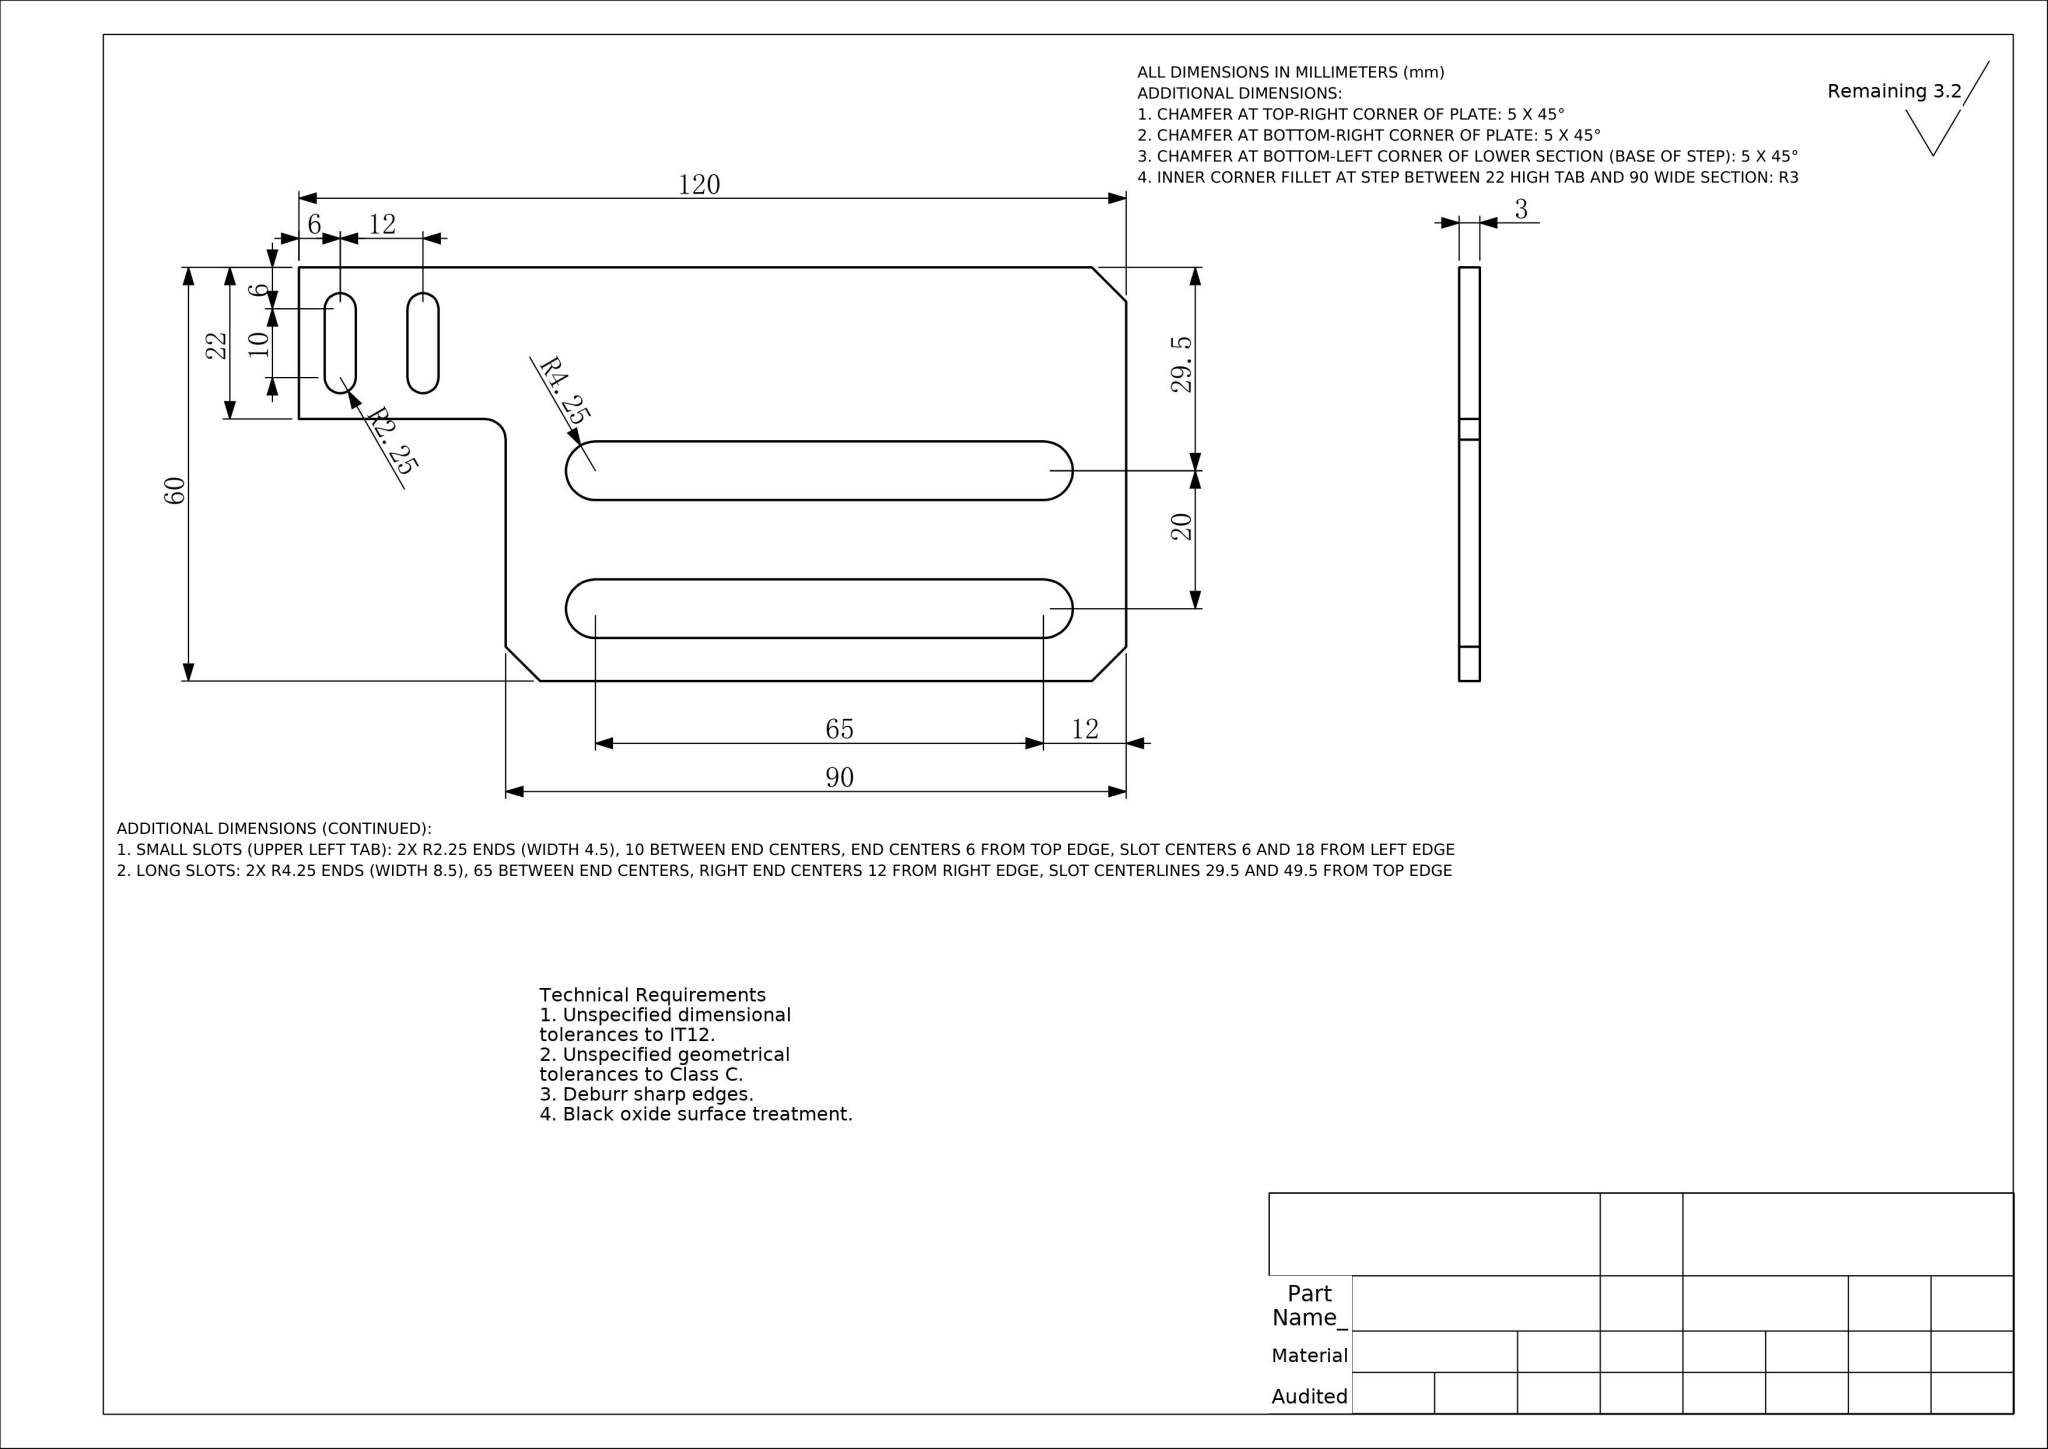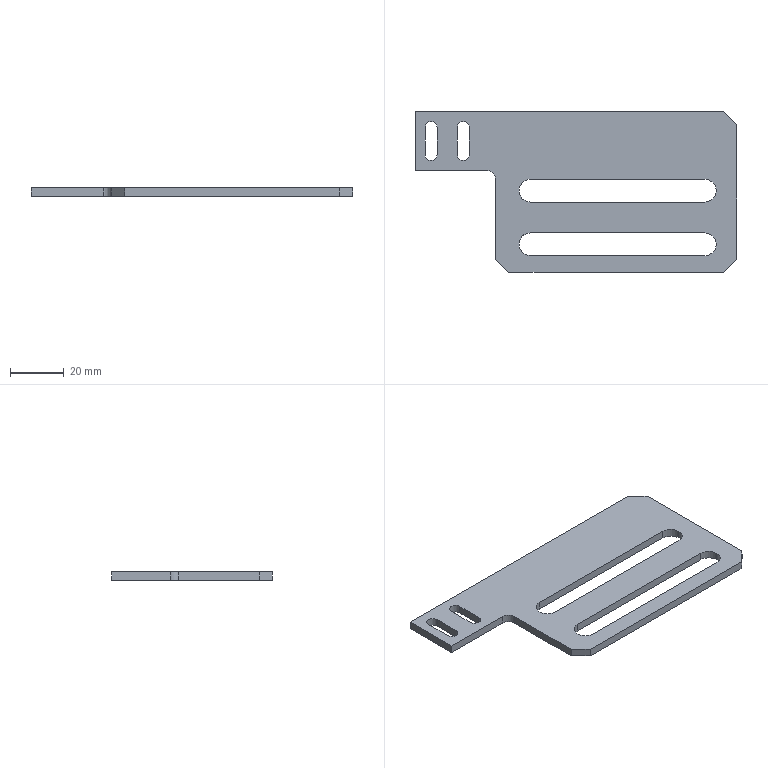Part | NX | mm | 1 solid | 30 faces | box 120 x 60 x 3 mm | volume 14052 mm3 | plane 19 | cylinder 11 | commonest cylinder face diameters 8.5 x6 4.5 x4 6 x1
STEP:
#1=COLOUR_RGB('',0.7961,0.8235,0.9373);
#2=FILL_AREA_STYLE_COLOUR('',#1);
#3=FILL_AREA_STYLE('',(#2));
#4=SURFACE_STYLE_FILL_AREA(#3);
#5=SURFACE_SIDE_STYLE('',(#4));
#6=SURFACE_STYLE_USAGE(.BOTH.,#5);
#7=PRESENTATION_STYLE_ASSIGNMENT((#6));
#8=CARTESIAN_POINT('',(108.,-45.25,-0.));
#9=VERTEX_POINT('',#8);
#10=CARTESIAN_POINT('',(112.25,-49.5,0.));
#11=VERTEX_POINT('',#10);
#12=CARTESIAN_POINT('',(108.,-49.5,0.));
#13=DIRECTION('',(0.,0.,-1.));
#14=DIRECTION('',(1.,0.,0.));
#15=AXIS2_PLACEMENT_3D('',#12,#13,#14);
#16=CIRCLE('',#15,4.25);
#17=EDGE_CURVE('',#9,#11,#16,.T.);
#18=ORIENTED_EDGE('',*,*,#17,.T.);
#19=CARTESIAN_POINT('',(112.25,-49.5,3.));
#20=VERTEX_POINT('',#19);
#21=CARTESIAN_POINT('',(112.25,-49.5,-0.001));
#22=DIRECTION('',(0.,0.,1.));
#23=VECTOR('',#22,1000.);
#24=LINE('',#21,#23);
#25=EDGE_CURVE('',#11,#20,#24,.T.);
#26=ORIENTED_EDGE('',*,*,#25,.T.);
#27=CARTESIAN_POINT('',(108.,-45.25,3.));
#28=VERTEX_POINT('',#27);
#29=CARTESIAN_POINT('',(108.,-49.5,3.));
#30=DIRECTION('',(0.,0.,1.));
#31=DIRECTION('',(-1.,0.,0.));
#32=AXIS2_PLACEMENT_3D('',#29,#30,#31);
#33=CIRCLE('',#32,4.25);
#34=EDGE_CURVE('',#20,#28,#33,.T.);
#35=ORIENTED_EDGE('',*,*,#34,.T.);
#36=CARTESIAN_POINT('',(108.,-45.25,-0.001));
#37=DIRECTION('',(0.,0.,1.));
#38=VECTOR('',#37,1000.);
#39=LINE('',#36,#38);
#40=EDGE_CURVE('',#9,#28,#39,.T.);
#41=ORIENTED_EDGE('',*,*,#40,.F.);
#42=EDGE_LOOP('',(#18,#26,#35,#41));
#43=FACE_OUTER_BOUND('',#42,.T.);
#44=CARTESIAN_POINT('',(108.,-49.5,-0.001));
#45=DIRECTION('',(0.,0.,1.));
#46=DIRECTION('',(1.,0.,0.));
#47=AXIS2_PLACEMENT_3D('',#44,#45,#46);
#48=CYLINDRICAL_SURFACE('',#47,4.25);
#49=ADVANCED_FACE('',(#43),#48,.F.);
#50=CARTESIAN_POINT('',(108.,-25.25,-0.));
#51=VERTEX_POINT('',#50);
#52=CARTESIAN_POINT('',(112.25,-29.5,0.));
#53=VERTEX_POINT('',#52);
#54=CARTESIAN_POINT('',(108.,-29.5,0.));
#55=DIRECTION('',(0.,0.,-1.));
#56=DIRECTION('',(1.,0.,0.));
#57=AXIS2_PLACEMENT_3D('',#54,#55,#56);
#58=CIRCLE('',#57,4.25);
#59=EDGE_CURVE('',#51,#53,#58,.T.);
#60=ORIENTED_EDGE('',*,*,#59,.T.);
#61=CARTESIAN_POINT('',(112.25,-29.5,3.));
#62=VERTEX_POINT('',#61);
#63=CARTESIAN_POINT('',(112.25,-29.5,-0.001));
#64=DIRECTION('',(0.,0.,1.));
#65=VECTOR('',#64,1000.);
#66=LINE('',#63,#65);
#67=EDGE_CURVE('',#53,#62,#66,.T.);
#68=ORIENTED_EDGE('',*,*,#67,.T.);
#69=CARTESIAN_POINT('',(108.,-25.25,3.));
#70=VERTEX_POINT('',#69);
#71=CARTESIAN_POINT('',(108.,-29.5,3.));
#72=DIRECTION('',(0.,0.,1.));
#73=DIRECTION('',(-1.,0.,0.));
#74=AXIS2_PLACEMENT_3D('',#71,#72,#73);
#75=CIRCLE('',#74,4.25);
#76=EDGE_CURVE('',#62,#70,#75,.T.);
#77=ORIENTED_EDGE('',*,*,#76,.T.);
#78=CARTESIAN_POINT('',(108.,-25.25,-0.001));
#79=DIRECTION('',(0.,0.,1.));
#80=VECTOR('',#79,1000.);
#81=LINE('',#78,#80);
#82=EDGE_CURVE('',#51,#70,#81,.T.);
#83=ORIENTED_EDGE('',*,*,#82,.F.);
#84=EDGE_LOOP('',(#60,#68,#77,#83));
#85=FACE_OUTER_BOUND('',#84,.T.);
#86=CARTESIAN_POINT('',(108.,-29.5,-0.001));
#87=DIRECTION('',(0.,0.,1.));
#88=DIRECTION('',(1.,0.,0.));
#89=AXIS2_PLACEMENT_3D('',#86,#87,#88);
#90=CYLINDRICAL_SURFACE('',#89,4.25);
#91=ADVANCED_FACE('',(#85),#90,.F.);
#92=CARTESIAN_POINT('',(0.,0.,0.));
#93=VERTEX_POINT('',#92);
#94=CARTESIAN_POINT('',(0.,-22.,0.));
#95=VERTEX_POINT('',#94);
#96=CARTESIAN_POINT('',(0.,0.,0.));
#97=DIRECTION('',(0.,-1.,0.));
#98=VECTOR('',#97,1000.);
#99=LINE('',#96,#98);
#100=EDGE_CURVE('',#93,#95,#99,.T.);
#101=ORIENTED_EDGE('',*,*,#100,.T.);
#102=CARTESIAN_POINT('',(0.,-22.,3.));
#103=VERTEX_POINT('',#102);
#104=CARTESIAN_POINT('',(0.,-22.,3.));
#105=DIRECTION('',(0.,0.,-1.));
#106=VECTOR('',#105,1000.);
#107=LINE('',#104,#106);
#108=EDGE_CURVE('',#103,#95,#107,.T.);
#109=ORIENTED_EDGE('',*,*,#108,.F.);
#110=CARTESIAN_POINT('',(0.,0.,3.));
#111=VERTEX_POINT('',#110);
#112=CARTESIAN_POINT('',(0.,0.,3.));
#113=DIRECTION('',(0.,-1.,0.));
#114=VECTOR('',#113,1000.);
#115=LINE('',#112,#114);
#116=EDGE_CURVE('',#111,#103,#115,.T.);
#117=ORIENTED_EDGE('',*,*,#116,.F.);
#118=CARTESIAN_POINT('',(0.,0.,3.));
#119=DIRECTION('',(0.,0.,-1.));
#120=VECTOR('',#119,1000.);
#121=LINE('',#118,#120);
#122=EDGE_CURVE('',#111,#93,#121,.T.);
#123=ORIENTED_EDGE('',*,*,#122,.T.);
#124=EDGE_LOOP('',(#101,#109,#117,#123));
#125=FACE_OUTER_BOUND('',#124,.T.);
#126=CARTESIAN_POINT('',(0.,0.,3.));
#127=DIRECTION('',(1.,0.,0.));
#128=DIRECTION('',(-0.,1.,0.));
#129=AXIS2_PLACEMENT_3D('',#126,#127,#128);
#130=PLANE('',#129);
#131=ADVANCED_FACE('',(#125),#130,.F.);
#132=CARTESIAN_POINT('',(27.,-22.,0.));
#133=VERTEX_POINT('',#132);
#134=CARTESIAN_POINT('',(0.,-22.,0.));
#135=DIRECTION('',(1.,-0.,0.));
#136=VECTOR('',#135,1000.);
#137=LINE('',#134,#136);
#138=EDGE_CURVE('',#95,#133,#137,.T.);
#139=ORIENTED_EDGE('',*,*,#138,.T.);
#140=CARTESIAN_POINT('',(27.,-22.,3.));
#141=VERTEX_POINT('',#140);
#142=CARTESIAN_POINT('',(27.,-22.,3.));
#143=DIRECTION('',(0.,0.,-1.));
#144=VECTOR('',#143,1000.);
#145=LINE('',#142,#144);
#146=EDGE_CURVE('',#141,#133,#145,.T.);
#147=ORIENTED_EDGE('',*,*,#146,.F.);
#148=CARTESIAN_POINT('',(0.,-22.,3.));
#149=DIRECTION('',(1.,-0.,0.));
#150=VECTOR('',#149,1000.);
#151=LINE('',#148,#150);
#152=EDGE_CURVE('',#103,#141,#151,.T.);
#153=ORIENTED_EDGE('',*,*,#152,.F.);
#154=ORIENTED_EDGE('',*,*,#108,.T.);
#155=EDGE_LOOP('',(#139,#147,#153,#154));
#156=FACE_OUTER_BOUND('',#155,.T.);
#157=CARTESIAN_POINT('',(0.,-22.,3.));
#158=DIRECTION('',(0.,1.,0.));
#159=DIRECTION('',(-1.,0.,0.));
#160=AXIS2_PLACEMENT_3D('',#157,#158,#159);
#161=PLANE('',#160);
#162=ADVANCED_FACE('',(#156),#161,.F.);
#163=CARTESIAN_POINT('',(30.,-25.,0.));
#164=VERTEX_POINT('',#163);
#165=CARTESIAN_POINT('',(27.,-25.,0.));
#166=DIRECTION('',(0.,0.,-1.));
#167=DIRECTION('',(1.,0.,0.));
#168=AXIS2_PLACEMENT_3D('',#165,#166,#167);
#169=CIRCLE('',#168,3.);
#170=EDGE_CURVE('',#133,#164,#169,.T.);
#171=ORIENTED_EDGE('',*,*,#170,.T.);
#172=CARTESIAN_POINT('',(30.,-25.,3.));
#173=VERTEX_POINT('',#172);
#174=CARTESIAN_POINT('',(30.,-25.,3.));
#175=DIRECTION('',(0.,0.,-1.));
#176=VECTOR('',#175,1000.);
#177=LINE('',#174,#176);
#178=EDGE_CURVE('',#173,#164,#177,.T.);
#179=ORIENTED_EDGE('',*,*,#178,.F.);
#180=CARTESIAN_POINT('',(27.,-25.,3.));
#181=DIRECTION('',(0.,0.,-1.));
#182=DIRECTION('',(1.,0.,0.));
#183=AXIS2_PLACEMENT_3D('',#180,#181,#182);
#184=CIRCLE('',#183,3.);
#185=EDGE_CURVE('',#141,#173,#184,.T.);
#186=ORIENTED_EDGE('',*,*,#185,.F.);
#187=ORIENTED_EDGE('',*,*,#146,.T.);
#188=EDGE_LOOP('',(#171,#179,#186,#187));
#189=FACE_OUTER_BOUND('',#188,.T.);
#190=CARTESIAN_POINT('',(27.,-25.,3.));
#191=DIRECTION('',(0.,0.,-1.));
#192=DIRECTION('',(-1.,0.,0.));
#193=AXIS2_PLACEMENT_3D('',#190,#191,#192);
#194=CYLINDRICAL_SURFACE('',#193,3.);
#195=ADVANCED_FACE('',(#189),#194,.F.);
#196=CARTESIAN_POINT('',(30.,-55.,0.));
#197=VERTEX_POINT('',#196);
#198=CARTESIAN_POINT('',(30.,-60.,0.));
#199=DIRECTION('',(0.,-1.,0.));
#200=VECTOR('',#199,1000.);
#201=LINE('',#198,#200);
#202=EDGE_CURVE('',#164,#197,#201,.T.);
#203=ORIENTED_EDGE('',*,*,#202,.T.);
#204=CARTESIAN_POINT('',(30.,-55.,3.));
#205=VERTEX_POINT('',#204);
#206=CARTESIAN_POINT('',(30.,-55.,3.));
#207=DIRECTION('',(0.,0.,1.));
#208=VECTOR('',#207,1000.);
#209=LINE('',#206,#208);
#210=EDGE_CURVE('',#197,#205,#209,.T.);
#211=ORIENTED_EDGE('',*,*,#210,.T.);
#212=CARTESIAN_POINT('',(30.,-60.,3.));
#213=DIRECTION('',(0.,-1.,0.));
#214=VECTOR('',#213,1000.);
#215=LINE('',#212,#214);
#216=EDGE_CURVE('',#173,#205,#215,.T.);
#217=ORIENTED_EDGE('',*,*,#216,.F.);
#218=ORIENTED_EDGE('',*,*,#178,.T.);
#219=EDGE_LOOP('',(#203,#211,#217,#218));
#220=FACE_OUTER_BOUND('',#219,.T.);
#221=CARTESIAN_POINT('',(30.,-60.,3.));
#222=DIRECTION('',(1.,0.,0.));
#223=DIRECTION('',(0.,0.,-1.));
#224=AXIS2_PLACEMENT_3D('',#221,#222,#223);
#225=PLANE('',#224);
#226=ADVANCED_FACE('',(#220),#225,.F.);
#227=CARTESIAN_POINT('',(35.,-60.,3.));
#228=VERTEX_POINT('',#227);
#229=CARTESIAN_POINT('',(115.,-60.,3.));
#230=VERTEX_POINT('',#229);
#231=CARTESIAN_POINT('',(30.,-60.,3.));
#232=DIRECTION('',(1.,0.,0.));
#233=VECTOR('',#232,1000.);
#234=LINE('',#231,#233);
#235=EDGE_CURVE('',#228,#230,#234,.T.);
#236=ORIENTED_EDGE('',*,*,#235,.F.);
#237=CARTESIAN_POINT('',(35.,-60.,0.));
#238=VERTEX_POINT('',#237);
#239=CARTESIAN_POINT('',(35.,-60.,3.));
#240=DIRECTION('',(0.,0.,-1.));
#241=VECTOR('',#240,1000.);
#242=LINE('',#239,#241);
#243=EDGE_CURVE('',#228,#238,#242,.T.);
#244=ORIENTED_EDGE('',*,*,#243,.T.);
#245=CARTESIAN_POINT('',(115.,-60.,0.));
#246=VERTEX_POINT('',#245);
#247=CARTESIAN_POINT('',(30.,-60.,0.));
#248=DIRECTION('',(1.,0.,0.));
#249=VECTOR('',#248,1000.);
#250=LINE('',#247,#249);
#251=EDGE_CURVE('',#238,#246,#250,.T.);
#252=ORIENTED_EDGE('',*,*,#251,.T.);
#253=CARTESIAN_POINT('',(115.,-60.,3.));
#254=DIRECTION('',(0.,0.,1.));
#255=VECTOR('',#254,1000.);
#256=LINE('',#253,#255);
#257=EDGE_CURVE('',#246,#230,#256,.T.);
#258=ORIENTED_EDGE('',*,*,#257,.T.);
#259=EDGE_LOOP('',(#236,#244,#252,#258));
#260=FACE_OUTER_BOUND('',#259,.T.);
#261=CARTESIAN_POINT('',(30.,-60.,3.));
#262=DIRECTION('',(0.,1.,0.));
#263=DIRECTION('',(0.,0.,1.));
#264=AXIS2_PLACEMENT_3D('',#261,#262,#263);
#265=PLANE('',#264);
#266=ADVANCED_FACE('',(#260),#265,.F.);
#267=CARTESIAN_POINT('',(120.,-55.,3.));
#268=VERTEX_POINT('',#267);
#269=CARTESIAN_POINT('',(120.,-5.,3.));
#270=VERTEX_POINT('',#269);
#271=CARTESIAN_POINT('',(120.,0.,3.));
#272=DIRECTION('',(-0.,1.,0.));
#273=VECTOR('',#272,1000.);
#274=LINE('',#271,#273);
#275=EDGE_CURVE('',#268,#270,#274,.T.);
#276=ORIENTED_EDGE('',*,*,#275,.F.);
#277=CARTESIAN_POINT('',(120.,-55.,0.));
#278=VERTEX_POINT('',#277);
#279=CARTESIAN_POINT('',(120.,-55.,3.));
#280=DIRECTION('',(0.,0.,-1.));
#281=VECTOR('',#280,1000.);
#282=LINE('',#279,#281);
#283=EDGE_CURVE('',#268,#278,#282,.T.);
#284=ORIENTED_EDGE('',*,*,#283,.T.);
#285=CARTESIAN_POINT('',(120.,-5.,0.));
#286=VERTEX_POINT('',#285);
#287=CARTESIAN_POINT('',(120.,0.,0.));
#288=DIRECTION('',(-0.,1.,0.));
#289=VECTOR('',#288,1000.);
#290=LINE('',#287,#289);
#291=EDGE_CURVE('',#278,#286,#290,.T.);
#292=ORIENTED_EDGE('',*,*,#291,.T.);
#293=CARTESIAN_POINT('',(120.,-5.,3.));
#294=DIRECTION('',(0.,0.,1.));
#295=VECTOR('',#294,1000.);
#296=LINE('',#293,#295);
#297=EDGE_CURVE('',#286,#270,#296,.T.);
#298=ORIENTED_EDGE('',*,*,#297,.T.);
#299=EDGE_LOOP('',(#276,#284,#292,#298));
#300=FACE_OUTER_BOUND('',#299,.T.);
#301=CARTESIAN_POINT('',(120.,0.,3.));
#302=DIRECTION('',(-1.,-0.,0.));
#303=DIRECTION('',(0.,-1.,0.));
#304=AXIS2_PLACEMENT_3D('',#301,#302,#303);
#305=PLANE('',#304);
#306=ADVANCED_FACE('',(#300),#305,.F.);
#307=CARTESIAN_POINT('',(115.,0.,3.));
#308=VERTEX_POINT('',#307);
#309=CARTESIAN_POINT('',(0.,0.,3.));
#310=DIRECTION('',(-1.,0.,0.));
#311=VECTOR('',#310,1000.);
#312=LINE('',#309,#311);
#313=EDGE_CURVE('',#308,#111,#312,.T.);
#314=ORIENTED_EDGE('',*,*,#313,.F.);
#315=CARTESIAN_POINT('',(115.,0.,0.));
#316=VERTEX_POINT('',#315);
#317=CARTESIAN_POINT('',(115.,0.,3.));
#318=DIRECTION('',(0.,0.,-1.));
#319=VECTOR('',#318,1000.);
#320=LINE('',#317,#319);
#321=EDGE_CURVE('',#308,#316,#320,.T.);
#322=ORIENTED_EDGE('',*,*,#321,.T.);
#323=CARTESIAN_POINT('',(0.,0.,0.));
#324=DIRECTION('',(-1.,0.,0.));
#325=VECTOR('',#324,1000.);
#326=LINE('',#323,#325);
#327=EDGE_CURVE('',#316,#93,#326,.T.);
#328=ORIENTED_EDGE('',*,*,#327,.T.);
#329=ORIENTED_EDGE('',*,*,#122,.F.);
#330=EDGE_LOOP('',(#314,#322,#328,#329));
#331=FACE_OUTER_BOUND('',#330,.T.);
#332=CARTESIAN_POINT('',(0.,0.,3.));
#333=DIRECTION('',(0.,-1.,0.));
#334=DIRECTION('',(0.,0.,-1.));
#335=AXIS2_PLACEMENT_3D('',#332,#333,#334);
#336=PLANE('',#335);
#337=ADVANCED_FACE('',(#331),#336,.F.);
#338=CARTESIAN_POINT('',(20.25,-6.,3.));
#339=VERTEX_POINT('',#338);
#340=CARTESIAN_POINT('',(15.75,-6.,3.));
#341=VERTEX_POINT('',#340);
#342=CARTESIAN_POINT('',(18.,-6.,3.));
#343=DIRECTION('',(0.,0.,1.));
#344=DIRECTION('',(-1.,0.,0.));
#345=AXIS2_PLACEMENT_3D('',#342,#343,#344);
#346=CIRCLE('',#345,2.25);
#347=EDGE_CURVE('',#339,#341,#346,.T.);
#348=ORIENTED_EDGE('',*,*,#347,.F.);
#349=CARTESIAN_POINT('',(20.25,-16.,3.));
#350=VERTEX_POINT('',#349);
#351=CARTESIAN_POINT('',(20.25,-6.,3.));
#352=DIRECTION('',(0.,1.,0.));
#353=VECTOR('',#352,1000.);
#354=LINE('',#351,#353);
#355=EDGE_CURVE('',#350,#339,#354,.T.);
#356=ORIENTED_EDGE('',*,*,#355,.F.);
#357=CARTESIAN_POINT('',(15.75,-16.,3.));
#358=VERTEX_POINT('',#357);
#359=CARTESIAN_POINT('',(18.,-16.,3.));
#360=DIRECTION('',(0.,0.,1.));
#361=DIRECTION('',(1.,0.,0.));
#362=AXIS2_PLACEMENT_3D('',#359,#360,#361);
#363=CIRCLE('',#362,2.25);
#364=EDGE_CURVE('',#358,#350,#363,.T.);
#365=ORIENTED_EDGE('',*,*,#364,.F.);
#366=CARTESIAN_POINT('',(15.75,-6.,3.));
#367=DIRECTION('',(-0.,-1.,0.));
#368=VECTOR('',#367,1000.);
#369=LINE('',#366,#368);
#370=EDGE_CURVE('',#341,#358,#369,.T.);
#371=ORIENTED_EDGE('',*,*,#370,.F.);
#372=EDGE_LOOP('',(#348,#356,#365,#371));
#373=FACE_BOUND('',#372,.T.);
#374=CARTESIAN_POINT('',(8.25,-6.,3.));
#375=VERTEX_POINT('',#374);
#376=CARTESIAN_POINT('',(3.75,-6.,3.));
#377=VERTEX_POINT('',#376);
#378=CARTESIAN_POINT('',(6.,-6.,3.));
#379=DIRECTION('',(0.,0.,1.));
#380=DIRECTION('',(-1.,0.,0.));
#381=AXIS2_PLACEMENT_3D('',#378,#379,#380);
#382=CIRCLE('',#381,2.25);
#383=EDGE_CURVE('',#375,#377,#382,.T.);
#384=ORIENTED_EDGE('',*,*,#383,.F.);
#385=CARTESIAN_POINT('',(8.25,-16.,3.));
#386=VERTEX_POINT('',#385);
#387=CARTESIAN_POINT('',(8.25,-6.,3.));
#388=DIRECTION('',(0.,1.,0.));
#389=VECTOR('',#388,1000.);
#390=LINE('',#387,#389);
#391=EDGE_CURVE('',#386,#375,#390,.T.);
#392=ORIENTED_EDGE('',*,*,#391,.F.);
#393=CARTESIAN_POINT('',(3.75,-16.,3.));
#394=VERTEX_POINT('',#393);
#395=CARTESIAN_POINT('',(6.,-16.,3.));
#396=DIRECTION('',(0.,0.,1.));
#397=DIRECTION('',(1.,0.,0.));
#398=AXIS2_PLACEMENT_3D('',#395,#396,#397);
#399=CIRCLE('',#398,2.25);
#400=EDGE_CURVE('',#394,#386,#399,.T.);
#401=ORIENTED_EDGE('',*,*,#400,.F.);
#402=CARTESIAN_POINT('',(3.75,-6.,3.));
#403=DIRECTION('',(0.,-1.,0.));
#404=VECTOR('',#403,1000.);
#405=LINE('',#402,#404);
#406=EDGE_CURVE('',#377,#394,#405,.T.);
#407=ORIENTED_EDGE('',*,*,#406,.F.);
#408=EDGE_LOOP('',(#384,#392,#401,#407));
#409=FACE_BOUND('',#408,.T.);
#410=CARTESIAN_POINT('',(43.,-45.25,3.));
#411=VERTEX_POINT('',#410);
#412=CARTESIAN_POINT('',(43.,-53.75,3.));
#413=VERTEX_POINT('',#412);
#414=CARTESIAN_POINT('',(43.,-49.5,3.));
#415=DIRECTION('',(0.,0.,1.));
#416=DIRECTION('',(1.,0.,0.));
#417=AXIS2_PLACEMENT_3D('',#414,#415,#416);
#418=CIRCLE('',#417,4.25);
#419=EDGE_CURVE('',#411,#413,#418,.T.);
#420=ORIENTED_EDGE('',*,*,#419,.F.);
#421=CARTESIAN_POINT('',(43.,-45.25,3.));
#422=DIRECTION('',(-1.,0.,0.));
#423=VECTOR('',#422,1000.);
#424=LINE('',#421,#423);
#425=EDGE_CURVE('',#28,#411,#424,.T.);
#426=ORIENTED_EDGE('',*,*,#425,.F.);
#427=ORIENTED_EDGE('',*,*,#34,.F.);
#428=CARTESIAN_POINT('',(108.,-53.75,3.));
#429=VERTEX_POINT('',#428);
#430=CARTESIAN_POINT('',(108.,-49.5,3.));
#431=DIRECTION('',(0.,0.,1.));
#432=DIRECTION('',(-1.,0.,0.));
#433=AXIS2_PLACEMENT_3D('',#430,#431,#432);
#434=CIRCLE('',#433,4.25);
#435=EDGE_CURVE('',#429,#20,#434,.T.);
#436=ORIENTED_EDGE('',*,*,#435,.F.);
#437=CARTESIAN_POINT('',(43.,-53.75,3.));
#438=DIRECTION('',(1.,0.,0.));
#439=VECTOR('',#438,1000.);
#440=LINE('',#437,#439);
#441=EDGE_CURVE('',#413,#429,#440,.T.);
#442=ORIENTED_EDGE('',*,*,#441,.F.);
#443=EDGE_LOOP('',(#420,#426,#427,#436,#442));
#444=FACE_BOUND('',#443,.T.);
#445=CARTESIAN_POINT('',(43.,-25.25,3.));
#446=VERTEX_POINT('',#445);
#447=CARTESIAN_POINT('',(43.,-33.75,3.));
#448=VERTEX_POINT('',#447);
#449=CARTESIAN_POINT('',(43.,-29.5,3.));
#450=DIRECTION('',(0.,0.,1.));
#451=DIRECTION('',(1.,0.,0.));
#452=AXIS2_PLACEMENT_3D('',#449,#450,#451);
#453=CIRCLE('',#452,4.25);
#454=EDGE_CURVE('',#446,#448,#453,.T.);
#455=ORIENTED_EDGE('',*,*,#454,.F.);
#456=CARTESIAN_POINT('',(43.,-25.25,3.));
#457=DIRECTION('',(-1.,0.,0.));
#458=VECTOR('',#457,1000.);
#459=LINE('',#456,#458);
#460=EDGE_CURVE('',#70,#446,#459,.T.);
#461=ORIENTED_EDGE('',*,*,#460,.F.);
#462=ORIENTED_EDGE('',*,*,#76,.F.);
#463=CARTESIAN_POINT('',(108.,-33.75,3.));
#464=VERTEX_POINT('',#463);
#465=CARTESIAN_POINT('',(108.,-29.5,3.));
#466=DIRECTION('',(0.,0.,1.));
#467=DIRECTION('',(-1.,0.,0.));
#468=AXIS2_PLACEMENT_3D('',#465,#466,#467);
#469=CIRCLE('',#468,4.25);
#470=EDGE_CURVE('',#464,#62,#469,.T.);
#471=ORIENTED_EDGE('',*,*,#470,.F.);
#472=CARTESIAN_POINT('',(43.,-33.75,3.));
#473=DIRECTION('',(1.,0.,0.));
#474=VECTOR('',#473,1000.);
#475=LINE('',#472,#474);
#476=EDGE_CURVE('',#448,#464,#475,.T.);
#477=ORIENTED_EDGE('',*,*,#476,.F.);
#478=EDGE_LOOP('',(#455,#461,#462,#471,#477));
#479=FACE_BOUND('',#478,.T.);
#480=ORIENTED_EDGE('',*,*,#216,.T.);
#481=CARTESIAN_POINT('',(13.5,-38.5,3.));
#482=DIRECTION('',(0.7071,-0.7071,0.));
#483=VECTOR('',#482,1000.);
#484=LINE('',#481,#483);
#485=EDGE_CURVE('',#205,#228,#484,.T.);
#486=ORIENTED_EDGE('',*,*,#485,.T.);
#487=ORIENTED_EDGE('',*,*,#235,.T.);
#488=CARTESIAN_POINT('',(88.5,-86.5,3.));
#489=DIRECTION('',(0.7071,0.7071,0.));
#490=VECTOR('',#489,1000.);
#491=LINE('',#488,#490);
#492=EDGE_CURVE('',#230,#268,#491,.T.);
#493=ORIENTED_EDGE('',*,*,#492,.T.);
#494=ORIENTED_EDGE('',*,*,#275,.T.);
#495=CARTESIAN_POINT('',(83.5,31.5,3.));
#496=DIRECTION('',(-0.7071,0.7071,0.));
#497=VECTOR('',#496,1000.);
#498=LINE('',#495,#497);
#499=EDGE_CURVE('',#270,#308,#498,.T.);
#500=ORIENTED_EDGE('',*,*,#499,.T.);
#501=ORIENTED_EDGE('',*,*,#313,.T.);
#502=ORIENTED_EDGE('',*,*,#116,.T.);
#503=ORIENTED_EDGE('',*,*,#152,.T.);
#504=ORIENTED_EDGE('',*,*,#185,.T.);
#505=EDGE_LOOP('',(#480,#486,#487,#493,#494,#500,#501,#502,#503,#504));
#506=FACE_OUTER_BOUND('',#505,.T.);
#507=CARTESIAN_POINT('',(27.,-25.,3.));
#508=DIRECTION('',(0.,0.,1.));
#509=DIRECTION('',(1.,0.,0.));
#510=AXIS2_PLACEMENT_3D('',#507,#508,#509);
#511=PLANE('',#510);
#512=ADVANCED_FACE('',(#373,#409,#444,#479,#506),#511,.T.);
#513=CARTESIAN_POINT('',(20.25,-6.,-0.));
#514=VERTEX_POINT('',#513);
#515=CARTESIAN_POINT('',(20.25,-16.,-0.));
#516=VERTEX_POINT('',#515);
#517=CARTESIAN_POINT('',(20.25,-6.,0.));
#518=DIRECTION('',(0.,-1.,0.));
#519=VECTOR('',#518,1000.);
#520=LINE('',#517,#519);
#521=EDGE_CURVE('',#514,#516,#520,.T.);
#522=ORIENTED_EDGE('',*,*,#521,.F.);
#523=CARTESIAN_POINT('',(15.75,-6.,0.));
#524=VERTEX_POINT('',#523);
#525=CARTESIAN_POINT('',(18.,-6.,0.));
#526=DIRECTION('',(0.,0.,-1.));
#527=DIRECTION('',(1.,0.,0.));
#528=AXIS2_PLACEMENT_3D('',#525,#526,#527);
#529=CIRCLE('',#528,2.25);
#530=EDGE_CURVE('',#524,#514,#529,.T.);
#531=ORIENTED_EDGE('',*,*,#530,.F.);
#532=CARTESIAN_POINT('',(15.75,-16.,0.));
#533=VERTEX_POINT('',#532);
#534=CARTESIAN_POINT('',(15.75,-6.,0.));
#535=DIRECTION('',(0.,1.,0.));
#536=VECTOR('',#535,1000.);
#537=LINE('',#534,#536);
#538=EDGE_CURVE('',#533,#524,#537,.T.);
#539=ORIENTED_EDGE('',*,*,#538,.F.);
#540=CARTESIAN_POINT('',(18.,-16.,0.));
#541=DIRECTION('',(0.,0.,-1.));
#542=DIRECTION('',(1.,0.,0.));
#543=AXIS2_PLACEMENT_3D('',#540,#541,#542);
#544=CIRCLE('',#543,2.25);
#545=EDGE_CURVE('',#516,#533,#544,.T.);
#546=ORIENTED_EDGE('',*,*,#545,.F.);
#547=EDGE_LOOP('',(#522,#531,#539,#546));
#548=FACE_BOUND('',#547,.T.);
#549=CARTESIAN_POINT('',(8.25,-6.,-0.));
#550=VERTEX_POINT('',#549);
#551=CARTESIAN_POINT('',(8.25,-16.,-0.));
#552=VERTEX_POINT('',#551);
#553=CARTESIAN_POINT('',(8.25,-6.,0.));
#554=DIRECTION('',(0.,-1.,0.));
#555=VECTOR('',#554,1000.);
#556=LINE('',#553,#555);
#557=EDGE_CURVE('',#550,#552,#556,.T.);
#558=ORIENTED_EDGE('',*,*,#557,.F.);
#559=CARTESIAN_POINT('',(3.75,-6.,0.));
#560=VERTEX_POINT('',#559);
#561=CARTESIAN_POINT('',(6.,-6.,0.));
#562=DIRECTION('',(0.,0.,-1.));
#563=DIRECTION('',(1.,0.,0.));
#564=AXIS2_PLACEMENT_3D('',#561,#562,#563);
#565=CIRCLE('',#564,2.25);
#566=EDGE_CURVE('',#560,#550,#565,.T.);
#567=ORIENTED_EDGE('',*,*,#566,.F.);
#568=CARTESIAN_POINT('',(3.75,-16.,0.));
#569=VERTEX_POINT('',#568);
#570=CARTESIAN_POINT('',(3.75,-6.,0.));
#571=DIRECTION('',(-0.,1.,0.));
#572=VECTOR('',#571,1000.);
#573=LINE('',#570,#572);
#574=EDGE_CURVE('',#569,#560,#573,.T.);
#575=ORIENTED_EDGE('',*,*,#574,.F.);
#576=CARTESIAN_POINT('',(6.,-16.,0.));
#577=DIRECTION('',(0.,0.,-1.));
#578=DIRECTION('',(1.,0.,0.));
#579=AXIS2_PLACEMENT_3D('',#576,#577,#578);
#580=CIRCLE('',#579,2.25);
#581=EDGE_CURVE('',#552,#569,#580,.T.);
#582=ORIENTED_EDGE('',*,*,#581,.F.);
#583=EDGE_LOOP('',(#558,#567,#575,#582));
#584=FACE_BOUND('',#583,.T.);
#585=CARTESIAN_POINT('',(43.,-45.25,-0.));
#586=VERTEX_POINT('',#585);
#587=CARTESIAN_POINT('',(43.,-45.25,0.));
#588=DIRECTION('',(1.,-0.,0.));
#589=VECTOR('',#588,1000.);
#590=LINE('',#587,#589);
#591=EDGE_CURVE('',#586,#9,#590,.T.);
#592=ORIENTED_EDGE('',*,*,#591,.F.);
#593=CARTESIAN_POINT('',(43.,-53.75,0.));
#594=VERTEX_POINT('',#593);
#595=CARTESIAN_POINT('',(43.,-49.5,0.));
#596=DIRECTION('',(0.,0.,-1.));
#597=DIRECTION('',(1.,0.,0.));
#598=AXIS2_PLACEMENT_3D('',#595,#596,#597);
#599=CIRCLE('',#598,4.25);
#600=EDGE_CURVE('',#594,#586,#599,.T.);
#601=ORIENTED_EDGE('',*,*,#600,.F.);
#602=CARTESIAN_POINT('',(108.,-53.75,0.));
#603=VERTEX_POINT('',#602);
#604=CARTESIAN_POINT('',(43.,-53.75,0.));
#605=DIRECTION('',(-1.,0.,0.));
#606=VECTOR('',#605,1000.);
#607=LINE('',#604,#606);
#608=EDGE_CURVE('',#603,#594,#607,.T.);
#609=ORIENTED_EDGE('',*,*,#608,.F.);
#610=CARTESIAN_POINT('',(108.,-49.5,0.));
#611=DIRECTION('',(0.,0.,-1.));
#612=DIRECTION('',(1.,0.,0.));
#613=AXIS2_PLACEMENT_3D('',#610,#611,#612);
#614=CIRCLE('',#613,4.25);
#615=EDGE_CURVE('',#11,#603,#614,.T.);
#616=ORIENTED_EDGE('',*,*,#615,.F.);
#617=ORIENTED_EDGE('',*,*,#17,.F.);
#618=EDGE_LOOP('',(#592,#601,#609,#616,#617));
#619=FACE_BOUND('',#618,.T.);
#620=CARTESIAN_POINT('',(43.,-25.25,-0.));
#621=VERTEX_POINT('',#620);
#622=CARTESIAN_POINT('',(43.,-25.25,0.));
#623=DIRECTION('',(1.,-0.,0.));
#624=VECTOR('',#623,1000.);
#625=LINE('',#622,#624);
#626=EDGE_CURVE('',#621,#51,#625,.T.);
#627=ORIENTED_EDGE('',*,*,#626,.F.);
#628=CARTESIAN_POINT('',(43.,-33.75,0.));
#629=VERTEX_POINT('',#628);
#630=CARTESIAN_POINT('',(43.,-29.5,0.));
#631=DIRECTION('',(0.,0.,-1.));
#632=DIRECTION('',(1.,0.,0.));
#633=AXIS2_PLACEMENT_3D('',#630,#631,#632);
#634=CIRCLE('',#633,4.25);
#635=EDGE_CURVE('',#629,#621,#634,.T.);
#636=ORIENTED_EDGE('',*,*,#635,.F.);
#637=CARTESIAN_POINT('',(108.,-33.75,0.));
#638=VERTEX_POINT('',#637);
#639=CARTESIAN_POINT('',(43.,-33.75,0.));
#640=DIRECTION('',(-1.,0.,0.));
#641=VECTOR('',#640,1000.);
#642=LINE('',#639,#641);
#643=EDGE_CURVE('',#638,#629,#642,.T.);
#644=ORIENTED_EDGE('',*,*,#643,.F.);
#645=CARTESIAN_POINT('',(108.,-29.5,0.));
#646=DIRECTION('',(0.,0.,-1.));
#647=DIRECTION('',(1.,0.,0.));
#648=AXIS2_PLACEMENT_3D('',#645,#646,#647);
#649=CIRCLE('',#648,4.25);
#650=EDGE_CURVE('',#53,#638,#649,.T.);
#651=ORIENTED_EDGE('',*,*,#650,.F.);
#652=ORIENTED_EDGE('',*,*,#59,.F.);
#653=EDGE_LOOP('',(#627,#636,#644,#651,#652));
#654=FACE_BOUND('',#653,.T.);
#655=ORIENTED_EDGE('',*,*,#251,.F.);
#656=CARTESIAN_POINT('',(35.,-60.,0.));
#657=DIRECTION('',(-0.7071,0.7071,0.));
#658=VECTOR('',#657,1000.);
#659=LINE('',#656,#658);
#660=EDGE_CURVE('',#238,#197,#659,.T.);
#661=ORIENTED_EDGE('',*,*,#660,.T.);
#662=ORIENTED_EDGE('',*,*,#202,.F.);
#663=ORIENTED_EDGE('',*,*,#170,.F.);
#664=ORIENTED_EDGE('',*,*,#138,.F.);
#665=ORIENTED_EDGE('',*,*,#100,.F.);
#666=ORIENTED_EDGE('',*,*,#327,.F.);
#667=CARTESIAN_POINT('',(115.,0.,0.));
#668=DIRECTION('',(0.7071,-0.7071,0.));
#669=VECTOR('',#668,1000.);
#670=LINE('',#667,#669);
#671=EDGE_CURVE('',#316,#286,#670,.T.);
#672=ORIENTED_EDGE('',*,*,#671,.T.);
#673=ORIENTED_EDGE('',*,*,#291,.F.);
#674=CARTESIAN_POINT('',(120.,-55.,0.));
#675=DIRECTION('',(-0.7071,-0.7071,0.));
#676=VECTOR('',#675,1000.);
#677=LINE('',#674,#676);
#678=EDGE_CURVE('',#278,#246,#677,.T.);
#679=ORIENTED_EDGE('',*,*,#678,.T.);
#680=EDGE_LOOP('',(#655,#661,#662,#663,#664,#665,#666,#672,#673,#679));
#681=FACE_OUTER_BOUND('',#680,.T.);
#682=CARTESIAN_POINT('',(27.,-25.,0.));
#683=DIRECTION('',(0.,0.,1.));
#684=DIRECTION('',(1.,0.,0.));
#685=AXIS2_PLACEMENT_3D('',#682,#683,#684);
#686=PLANE('',#685);
#687=ADVANCED_FACE('',(#548,#584,#619,#654,#681),#686,.F.);
#688=ORIENTED_EDGE('',*,*,#635,.T.);
#689=CARTESIAN_POINT('',(43.,-25.25,-0.001));
#690=DIRECTION('',(0.,0.,1.));
#691=VECTOR('',#690,1000.);
#692=LINE('',#689,#691);
#693=EDGE_CURVE('',#621,#446,#692,.T.);
#694=ORIENTED_EDGE('',*,*,#693,.T.);
#695=ORIENTED_EDGE('',*,*,#454,.T.);
#696=CARTESIAN_POINT('',(43.,-33.75,-0.001));
#697=DIRECTION('',(0.,0.,1.));
#698=VECTOR('',#697,1000.);
#699=LINE('',#696,#698);
#700=EDGE_CURVE('',#629,#448,#699,.T.);
#701=ORIENTED_EDGE('',*,*,#700,.F.);
#702=EDGE_LOOP('',(#688,#694,#695,#701));
#703=FACE_OUTER_BOUND('',#702,.T.);
#704=CARTESIAN_POINT('',(43.,-29.5,-0.001));
#705=DIRECTION('',(0.,0.,1.));
#706=DIRECTION('',(1.,0.,0.));
#707=AXIS2_PLACEMENT_3D('',#704,#705,#706);
#708=CYLINDRICAL_SURFACE('',#707,4.25);
#709=ADVANCED_FACE('',(#703),#708,.F.);
#710=ORIENTED_EDGE('',*,*,#626,.T.);
#711=ORIENTED_EDGE('',*,*,#82,.T.);
#712=ORIENTED_EDGE('',*,*,#460,.T.);
#713=ORIENTED_EDGE('',*,*,#693,.F.);
#714=EDGE_LOOP('',(#710,#711,#712,#713));
#715=FACE_OUTER_BOUND('',#714,.T.);
#716=CARTESIAN_POINT('',(43.,-25.25,-0.001));
#717=DIRECTION('',(0.,1.,0.));
#718=DIRECTION('',(-1.,0.,0.));
#719=AXIS2_PLACEMENT_3D('',#716,#717,#718);
#720=PLANE('',#719);
#721=ADVANCED_FACE('',(#715),#720,.F.);
#722=ORIENTED_EDGE('',*,*,#67,.F.);
#723=ORIENTED_EDGE('',*,*,#650,.T.);
#724=CARTESIAN_POINT('',(108.,-33.75,-0.001));
#725=DIRECTION('',(0.,0.,1.));
#726=VECTOR('',#725,1000.);
#727=LINE('',#724,#726);
#728=EDGE_CURVE('',#638,#464,#727,.T.);
#729=ORIENTED_EDGE('',*,*,#728,.T.);
#730=ORIENTED_EDGE('',*,*,#470,.T.);
#731=EDGE_LOOP('',(#722,#723,#729,#730));
#732=FACE_OUTER_BOUND('',#731,.T.);
#733=CARTESIAN_POINT('',(108.,-29.5,-0.001));
#734=DIRECTION('',(0.,0.,1.));
#735=DIRECTION('',(1.,0.,0.));
#736=AXIS2_PLACEMENT_3D('',#733,#734,#735);
#737=CYLINDRICAL_SURFACE('',#736,4.25);
#738=ADVANCED_FACE('',(#732),#737,.F.);
#739=ORIENTED_EDGE('',*,*,#643,.T.);
#740=ORIENTED_EDGE('',*,*,#700,.T.);
#741=ORIENTED_EDGE('',*,*,#476,.T.);
#742=ORIENTED_EDGE('',*,*,#728,.F.);
#743=EDGE_LOOP('',(#739,#740,#741,#742));
#744=FACE_OUTER_BOUND('',#743,.T.);
#745=CARTESIAN_POINT('',(43.,-33.75,-0.001));
#746=DIRECTION('',(0.,-1.,0.));
#747=DIRECTION('',(0.,0.,-1.));
#748=AXIS2_PLACEMENT_3D('',#745,#746,#747);
#749=PLANE('',#748);
#750=ADVANCED_FACE('',(#744),#749,.F.);
#751=ORIENTED_EDGE('',*,*,#600,.T.);
#752=CARTESIAN_POINT('',(43.,-45.25,-0.001));
#753=DIRECTION('',(0.,0.,1.));
#754=VECTOR('',#753,1000.);
#755=LINE('',#752,#754);
#756=EDGE_CURVE('',#586,#411,#755,.T.);
#757=ORIENTED_EDGE('',*,*,#756,.T.);
#758=ORIENTED_EDGE('',*,*,#419,.T.);
#759=CARTESIAN_POINT('',(43.,-53.75,-0.001));
#760=DIRECTION('',(0.,0.,1.));
#761=VECTOR('',#760,1000.);
#762=LINE('',#759,#761);
#763=EDGE_CURVE('',#594,#413,#762,.T.);
#764=ORIENTED_EDGE('',*,*,#763,.F.);
#765=EDGE_LOOP('',(#751,#757,#758,#764));
#766=FACE_OUTER_BOUND('',#765,.T.);
#767=CARTESIAN_POINT('',(43.,-49.5,-0.001));
#768=DIRECTION('',(0.,0.,1.));
#769=DIRECTION('',(1.,0.,0.));
#770=AXIS2_PLACEMENT_3D('',#767,#768,#769);
#771=CYLINDRICAL_SURFACE('',#770,4.25);
#772=ADVANCED_FACE('',(#766),#771,.F.);
#773=ORIENTED_EDGE('',*,*,#591,.T.);
#774=ORIENTED_EDGE('',*,*,#40,.T.);
#775=ORIENTED_EDGE('',*,*,#425,.T.);
#776=ORIENTED_EDGE('',*,*,#756,.F.);
#777=EDGE_LOOP('',(#773,#774,#775,#776));
#778=FACE_OUTER_BOUND('',#777,.T.);
#779=CARTESIAN_POINT('',(43.,-45.25,-0.001));
#780=DIRECTION('',(0.,1.,0.));
#781=DIRECTION('',(-1.,0.,0.));
#782=AXIS2_PLACEMENT_3D('',#779,#780,#781);
#783=PLANE('',#782);
#784=ADVANCED_FACE('',(#778),#783,.F.);
#785=ORIENTED_EDGE('',*,*,#25,.F.);
#786=ORIENTED_EDGE('',*,*,#615,.T.);
#787=CARTESIAN_POINT('',(108.,-53.75,-0.001));
#788=DIRECTION('',(0.,0.,1.));
#789=VECTOR('',#788,1000.);
#790=LINE('',#787,#789);
#791=EDGE_CURVE('',#603,#429,#790,.T.);
#792=ORIENTED_EDGE('',*,*,#791,.T.);
#793=ORIENTED_EDGE('',*,*,#435,.T.);
#794=EDGE_LOOP('',(#785,#786,#792,#793));
#795=FACE_OUTER_BOUND('',#794,.T.);
#796=CARTESIAN_POINT('',(108.,-49.5,-0.001));
#797=DIRECTION('',(0.,0.,1.));
#798=DIRECTION('',(1.,0.,0.));
#799=AXIS2_PLACEMENT_3D('',#796,#797,#798);
#800=CYLINDRICAL_SURFACE('',#799,4.25);
#801=ADVANCED_FACE('',(#795),#800,.F.);
#802=ORIENTED_EDGE('',*,*,#608,.T.);
#803=ORIENTED_EDGE('',*,*,#763,.T.);
#804=ORIENTED_EDGE('',*,*,#441,.T.);
#805=ORIENTED_EDGE('',*,*,#791,.F.);
#806=EDGE_LOOP('',(#802,#803,#804,#805));
#807=FACE_OUTER_BOUND('',#806,.T.);
#808=CARTESIAN_POINT('',(43.,-53.75,-0.001));
#809=DIRECTION('',(0.,-1.,0.));
#810=DIRECTION('',(0.,0.,-1.));
#811=AXIS2_PLACEMENT_3D('',#808,#809,#810);
#812=PLANE('',#811);
#813=ADVANCED_FACE('',(#807),#812,.F.);
#814=ORIENTED_EDGE('',*,*,#566,.T.);
#815=CARTESIAN_POINT('',(8.25,-6.,-0.001));
#816=DIRECTION('',(0.,0.,1.));
#817=VECTOR('',#816,1000.);
#818=LINE('',#815,#817);
#819=EDGE_CURVE('',#550,#375,#818,.T.);
#820=ORIENTED_EDGE('',*,*,#819,.T.);
#821=ORIENTED_EDGE('',*,*,#383,.T.);
#822=CARTESIAN_POINT('',(3.75,-6.,-0.001));
#823=DIRECTION('',(0.,0.,1.));
#824=VECTOR('',#823,1000.);
#825=LINE('',#822,#824);
#826=EDGE_CURVE('',#560,#377,#825,.T.);
#827=ORIENTED_EDGE('',*,*,#826,.F.);
#828=EDGE_LOOP('',(#814,#820,#821,#827));
#829=FACE_OUTER_BOUND('',#828,.T.);
#830=CARTESIAN_POINT('',(6.,-6.,-0.001));
#831=DIRECTION('',(0.,0.,1.));
#832=DIRECTION('',(1.,0.,0.));
#833=AXIS2_PLACEMENT_3D('',#830,#831,#832);
#834=CYLINDRICAL_SURFACE('',#833,2.25);
#835=ADVANCED_FACE('',(#829),#834,.F.);
#836=ORIENTED_EDGE('',*,*,#557,.T.);
#837=CARTESIAN_POINT('',(8.25,-16.,-0.001));
#838=DIRECTION('',(0.,0.,1.));
#839=VECTOR('',#838,1000.);
#840=LINE('',#837,#839);
#841=EDGE_CURVE('',#552,#386,#840,.T.);
#842=ORIENTED_EDGE('',*,*,#841,.T.);
#843=ORIENTED_EDGE('',*,*,#391,.T.);
#844=ORIENTED_EDGE('',*,*,#819,.F.);
#845=EDGE_LOOP('',(#836,#842,#843,#844));
#846=FACE_OUTER_BOUND('',#845,.T.);
#847=CARTESIAN_POINT('',(8.25,-6.,-0.001));
#848=DIRECTION('',(1.,0.,0.));
#849=DIRECTION('',(0.,0.,-1.));
#850=AXIS2_PLACEMENT_3D('',#847,#848,#849);
#851=PLANE('',#850);
#852=ADVANCED_FACE('',(#846),#851,.F.);
#853=ORIENTED_EDGE('',*,*,#581,.T.);
#854=CARTESIAN_POINT('',(3.75,-16.,-0.001));
#855=DIRECTION('',(0.,0.,1.));
#856=VECTOR('',#855,1000.);
#857=LINE('',#854,#856);
#858=EDGE_CURVE('',#569,#394,#857,.T.);
#859=ORIENTED_EDGE('',*,*,#858,.T.);
#860=ORIENTED_EDGE('',*,*,#400,.T.);
#861=ORIENTED_EDGE('',*,*,#841,.F.);
#862=EDGE_LOOP('',(#853,#859,#860,#861));
#863=FACE_OUTER_BOUND('',#862,.T.);
#864=CARTESIAN_POINT('',(6.,-16.,-0.001));
#865=DIRECTION('',(0.,0.,1.));
#866=DIRECTION('',(1.,0.,0.));
#867=AXIS2_PLACEMENT_3D('',#864,#865,#866);
#868=CYLINDRICAL_SURFACE('',#867,2.25);
#869=ADVANCED_FACE('',(#863),#868,.F.);
#870=ORIENTED_EDGE('',*,*,#574,.T.);
#871=ORIENTED_EDGE('',*,*,#826,.T.);
#872=ORIENTED_EDGE('',*,*,#406,.T.);
#873=ORIENTED_EDGE('',*,*,#858,.F.);
#874=EDGE_LOOP('',(#870,#871,#872,#873));
#875=FACE_OUTER_BOUND('',#874,.T.);
#876=CARTESIAN_POINT('',(3.75,-6.,-0.001));
#877=DIRECTION('',(-1.,-0.,0.));
#878=DIRECTION('',(0.,-1.,0.));
#879=AXIS2_PLACEMENT_3D('',#876,#877,#878);
#880=PLANE('',#879);
#881=ADVANCED_FACE('',(#875),#880,.F.);
#882=ORIENTED_EDGE('',*,*,#530,.T.);
#883=CARTESIAN_POINT('',(20.25,-6.,-0.001));
#884=DIRECTION('',(0.,0.,1.));
#885=VECTOR('',#884,1000.);
#886=LINE('',#883,#885);
#887=EDGE_CURVE('',#514,#339,#886,.T.);
#888=ORIENTED_EDGE('',*,*,#887,.T.);
#889=ORIENTED_EDGE('',*,*,#347,.T.);
#890=CARTESIAN_POINT('',(15.75,-6.,-0.001));
#891=DIRECTION('',(0.,0.,1.));
#892=VECTOR('',#891,1000.);
#893=LINE('',#890,#892);
#894=EDGE_CURVE('',#524,#341,#893,.T.);
#895=ORIENTED_EDGE('',*,*,#894,.F.);
#896=EDGE_LOOP('',(#882,#888,#889,#895));
#897=FACE_OUTER_BOUND('',#896,.T.);
#898=CARTESIAN_POINT('',(18.,-6.,-0.001));
#899=DIRECTION('',(0.,0.,1.));
#900=DIRECTION('',(1.,0.,0.));
#901=AXIS2_PLACEMENT_3D('',#898,#899,#900);
#902=CYLINDRICAL_SURFACE('',#901,2.25);
#903=ADVANCED_FACE('',(#897),#902,.F.);
#904=ORIENTED_EDGE('',*,*,#521,.T.);
#905=CARTESIAN_POINT('',(20.25,-16.,-0.001));
#906=DIRECTION('',(0.,0.,1.));
#907=VECTOR('',#906,1000.);
#908=LINE('',#905,#907);
#909=EDGE_CURVE('',#516,#350,#908,.T.);
#910=ORIENTED_EDGE('',*,*,#909,.T.);
#911=ORIENTED_EDGE('',*,*,#355,.T.);
#912=ORIENTED_EDGE('',*,*,#887,.F.);
#913=EDGE_LOOP('',(#904,#910,#911,#912));
#914=FACE_OUTER_BOUND('',#913,.T.);
#915=CARTESIAN_POINT('',(20.25,-6.,-0.001));
#916=DIRECTION('',(1.,0.,0.));
#917=DIRECTION('',(0.,0.,-1.));
#918=AXIS2_PLACEMENT_3D('',#915,#916,#917);
#919=PLANE('',#918);
#920=ADVANCED_FACE('',(#914),#919,.F.);
#921=ORIENTED_EDGE('',*,*,#545,.T.);
#922=CARTESIAN_POINT('',(15.75,-16.,-0.001));
#923=DIRECTION('',(0.,0.,1.));
#924=VECTOR('',#923,1000.);
#925=LINE('',#922,#924);
#926=EDGE_CURVE('',#533,#358,#925,.T.);
#927=ORIENTED_EDGE('',*,*,#926,.T.);
#928=ORIENTED_EDGE('',*,*,#364,.T.);
#929=ORIENTED_EDGE('',*,*,#909,.F.);
#930=EDGE_LOOP('',(#921,#927,#928,#929));
#931=FACE_OUTER_BOUND('',#930,.T.);
#932=CARTESIAN_POINT('',(18.,-16.,-0.001));
#933=DIRECTION('',(0.,0.,1.));
#934=DIRECTION('',(1.,0.,0.));
#935=AXIS2_PLACEMENT_3D('',#932,#933,#934);
#936=CYLINDRICAL_SURFACE('',#935,2.25);
#937=ADVANCED_FACE('',(#931),#936,.F.);
#938=ORIENTED_EDGE('',*,*,#538,.T.);
#939=ORIENTED_EDGE('',*,*,#894,.T.);
#940=ORIENTED_EDGE('',*,*,#370,.T.);
#941=ORIENTED_EDGE('',*,*,#926,.F.);
#942=EDGE_LOOP('',(#938,#939,#940,#941));
#943=FACE_OUTER_BOUND('',#942,.T.);
#944=CARTESIAN_POINT('',(15.75,-6.,-0.001));
#945=DIRECTION('',(-1.,0.,0.));
#946=DIRECTION('',(-0.,-1.,0.));
#947=AXIS2_PLACEMENT_3D('',#944,#945,#946);
#948=PLANE('',#947);
#949=ADVANCED_FACE('',(#943),#948,.F.);
#950=ORIENTED_EDGE('',*,*,#485,.F.);
#951=ORIENTED_EDGE('',*,*,#210,.F.);
#952=ORIENTED_EDGE('',*,*,#660,.F.);
#953=ORIENTED_EDGE('',*,*,#243,.F.);
#954=EDGE_LOOP('',(#950,#951,#952,#953));
#955=FACE_OUTER_BOUND('',#954,.T.);
#956=CARTESIAN_POINT('',(35.,-60.,3.));
#957=DIRECTION('',(0.7071,0.7071,0.));
#958=DIRECTION('',(-0.7071,0.7071,0.));
#959=AXIS2_PLACEMENT_3D('',#956,#957,#958);
#960=PLANE('',#959);
#961=ADVANCED_FACE('',(#955),#960,.F.);
#962=ORIENTED_EDGE('',*,*,#492,.F.);
#963=ORIENTED_EDGE('',*,*,#257,.F.);
#964=ORIENTED_EDGE('',*,*,#678,.F.);
#965=ORIENTED_EDGE('',*,*,#283,.F.);
#966=EDGE_LOOP('',(#962,#963,#964,#965));
#967=FACE_OUTER_BOUND('',#966,.T.);
#968=CARTESIAN_POINT('',(120.,-55.,3.));
#969=DIRECTION('',(-0.7071,0.7071,0.));
#970=DIRECTION('',(-0.7071,-0.7071,0.));
#971=AXIS2_PLACEMENT_3D('',#968,#969,#970);
#972=PLANE('',#971);
#973=ADVANCED_FACE('',(#967),#972,.F.);
#974=ORIENTED_EDGE('',*,*,#499,.F.);
#975=ORIENTED_EDGE('',*,*,#297,.F.);
#976=ORIENTED_EDGE('',*,*,#671,.F.);
#977=ORIENTED_EDGE('',*,*,#321,.F.);
#978=EDGE_LOOP('',(#974,#975,#976,#977));
#979=FACE_OUTER_BOUND('',#978,.T.);
#980=CARTESIAN_POINT('',(115.,0.,3.));
#981=DIRECTION('',(-0.7071,-0.7071,0.));
#982=DIRECTION('',(0.7071,-0.7071,0.));
#983=AXIS2_PLACEMENT_3D('',#980,#981,#982);
#984=PLANE('',#983);
#985=ADVANCED_FACE('',(#979),#984,.F.);
#986=CLOSED_SHELL('',(#49,#91,#131,#162,#195,#226,#266,#306,#337,#512,#687,#709,#721,#738,#750,#772,#784,#801,#813,#835,#852,#869,#881,#903,#920,#937,#949,#961,#973,#985));
#987=MANIFOLD_SOLID_BREP('',#986);
#988=STYLED_ITEM('',(#7),#987);
#989=(LENGTH_UNIT()NAMED_UNIT(*)SI_UNIT(.MILLI.,.METRE.));
#990=UNCERTAINTY_MEASURE_WITH_UNIT(LENGTH_MEASURE(0.00001),#989,'','');
#991=(NAMED_UNIT(*)PLANE_ANGLE_UNIT()SI_UNIT($,.RADIAN.));
#992=(NAMED_UNIT(*)SI_UNIT($,.STERADIAN.)SOLID_ANGLE_UNIT());
#993=(GEOMETRIC_REPRESENTATION_CONTEXT(3)GLOBAL_UNCERTAINTY_ASSIGNED_CONTEXT((#990))GLOBAL_UNIT_ASSIGNED_CONTEXT((#989,#991,#992))REPRESENTATION_CONTEXT('',''));
#994=MECHANICAL_DESIGN_GEOMETRIC_PRESENTATION_REPRESENTATION('',(#988),#993);
#995=PRESENTATION_LAYER_ASSIGNMENT('','',(#988));
#996=COLOUR_RGB('',0.7961,0.8235,0.9373);
#997=FILL_AREA_STYLE_COLOUR('',#996);
#998=FILL_AREA_STYLE('',(#997));
#999=SURFACE_STYLE_FILL_AREA(#998);
#1000=SURFACE_SIDE_STYLE('',(#999));
#1001=SURFACE_STYLE_USAGE(.BOTH.,#1000);
#1002=PRESENTATION_STYLE_ASSIGNMENT((#1001));
#1003=CARTESIAN_POINT('',(0.,0.,0.));
#1004=DIRECTION('',(0.,0.,1.));
#1005=DIRECTION('',(1.,0.,0.));
#1006=AXIS2_PLACEMENT_3D('',#1003,#1004,#1005);
#1007=(LENGTH_UNIT()NAMED_UNIT(*)SI_UNIT(.MILLI.,.METRE.));
#1008=UNCERTAINTY_MEASURE_WITH_UNIT(LENGTH_MEASURE(0.00001),#1007,'','');
#1009=(NAMED_UNIT(*)PLANE_ANGLE_UNIT()SI_UNIT($,.RADIAN.));
#1010=(NAMED_UNIT(*)SI_UNIT($,.STERADIAN.)SOLID_ANGLE_UNIT());
#1011=(GEOMETRIC_REPRESENTATION_CONTEXT(3)GLOBAL_UNCERTAINTY_ASSIGNED_CONTEXT((#1008))GLOBAL_UNIT_ASSIGNED_CONTEXT((#1007,#1009,#1010))REPRESENTATION_CONTEXT('',''));
#1012=ADVANCED_BREP_SHAPE_REPRESENTATION('',(#987,#1006),#1011);
#1013=STYLED_ITEM('',(#1002),#1012);
#1014=(LENGTH_UNIT()NAMED_UNIT(*)SI_UNIT(.MILLI.,.METRE.));
#1015=UNCERTAINTY_MEASURE_WITH_UNIT(LENGTH_MEASURE(0.00001),#1014,'','');
#1016=(NAMED_UNIT(*)PLANE_ANGLE_UNIT()SI_UNIT($,.RADIAN.));
#1017=(NAMED_UNIT(*)SI_UNIT($,.STERADIAN.)SOLID_ANGLE_UNIT());
#1018=(GEOMETRIC_REPRESENTATION_CONTEXT(3)GLOBAL_UNCERTAINTY_ASSIGNED_CONTEXT((#1015))GLOBAL_UNIT_ASSIGNED_CONTEXT((#1014,#1016,#1017))REPRESENTATION_CONTEXT('',''));
#1019=MECHANICAL_DESIGN_GEOMETRIC_PRESENTATION_REPRESENTATION('',(#1013),#1018);
#1020=PRESENTATION_LAYER_ASSIGNMENT('','',(#1013));